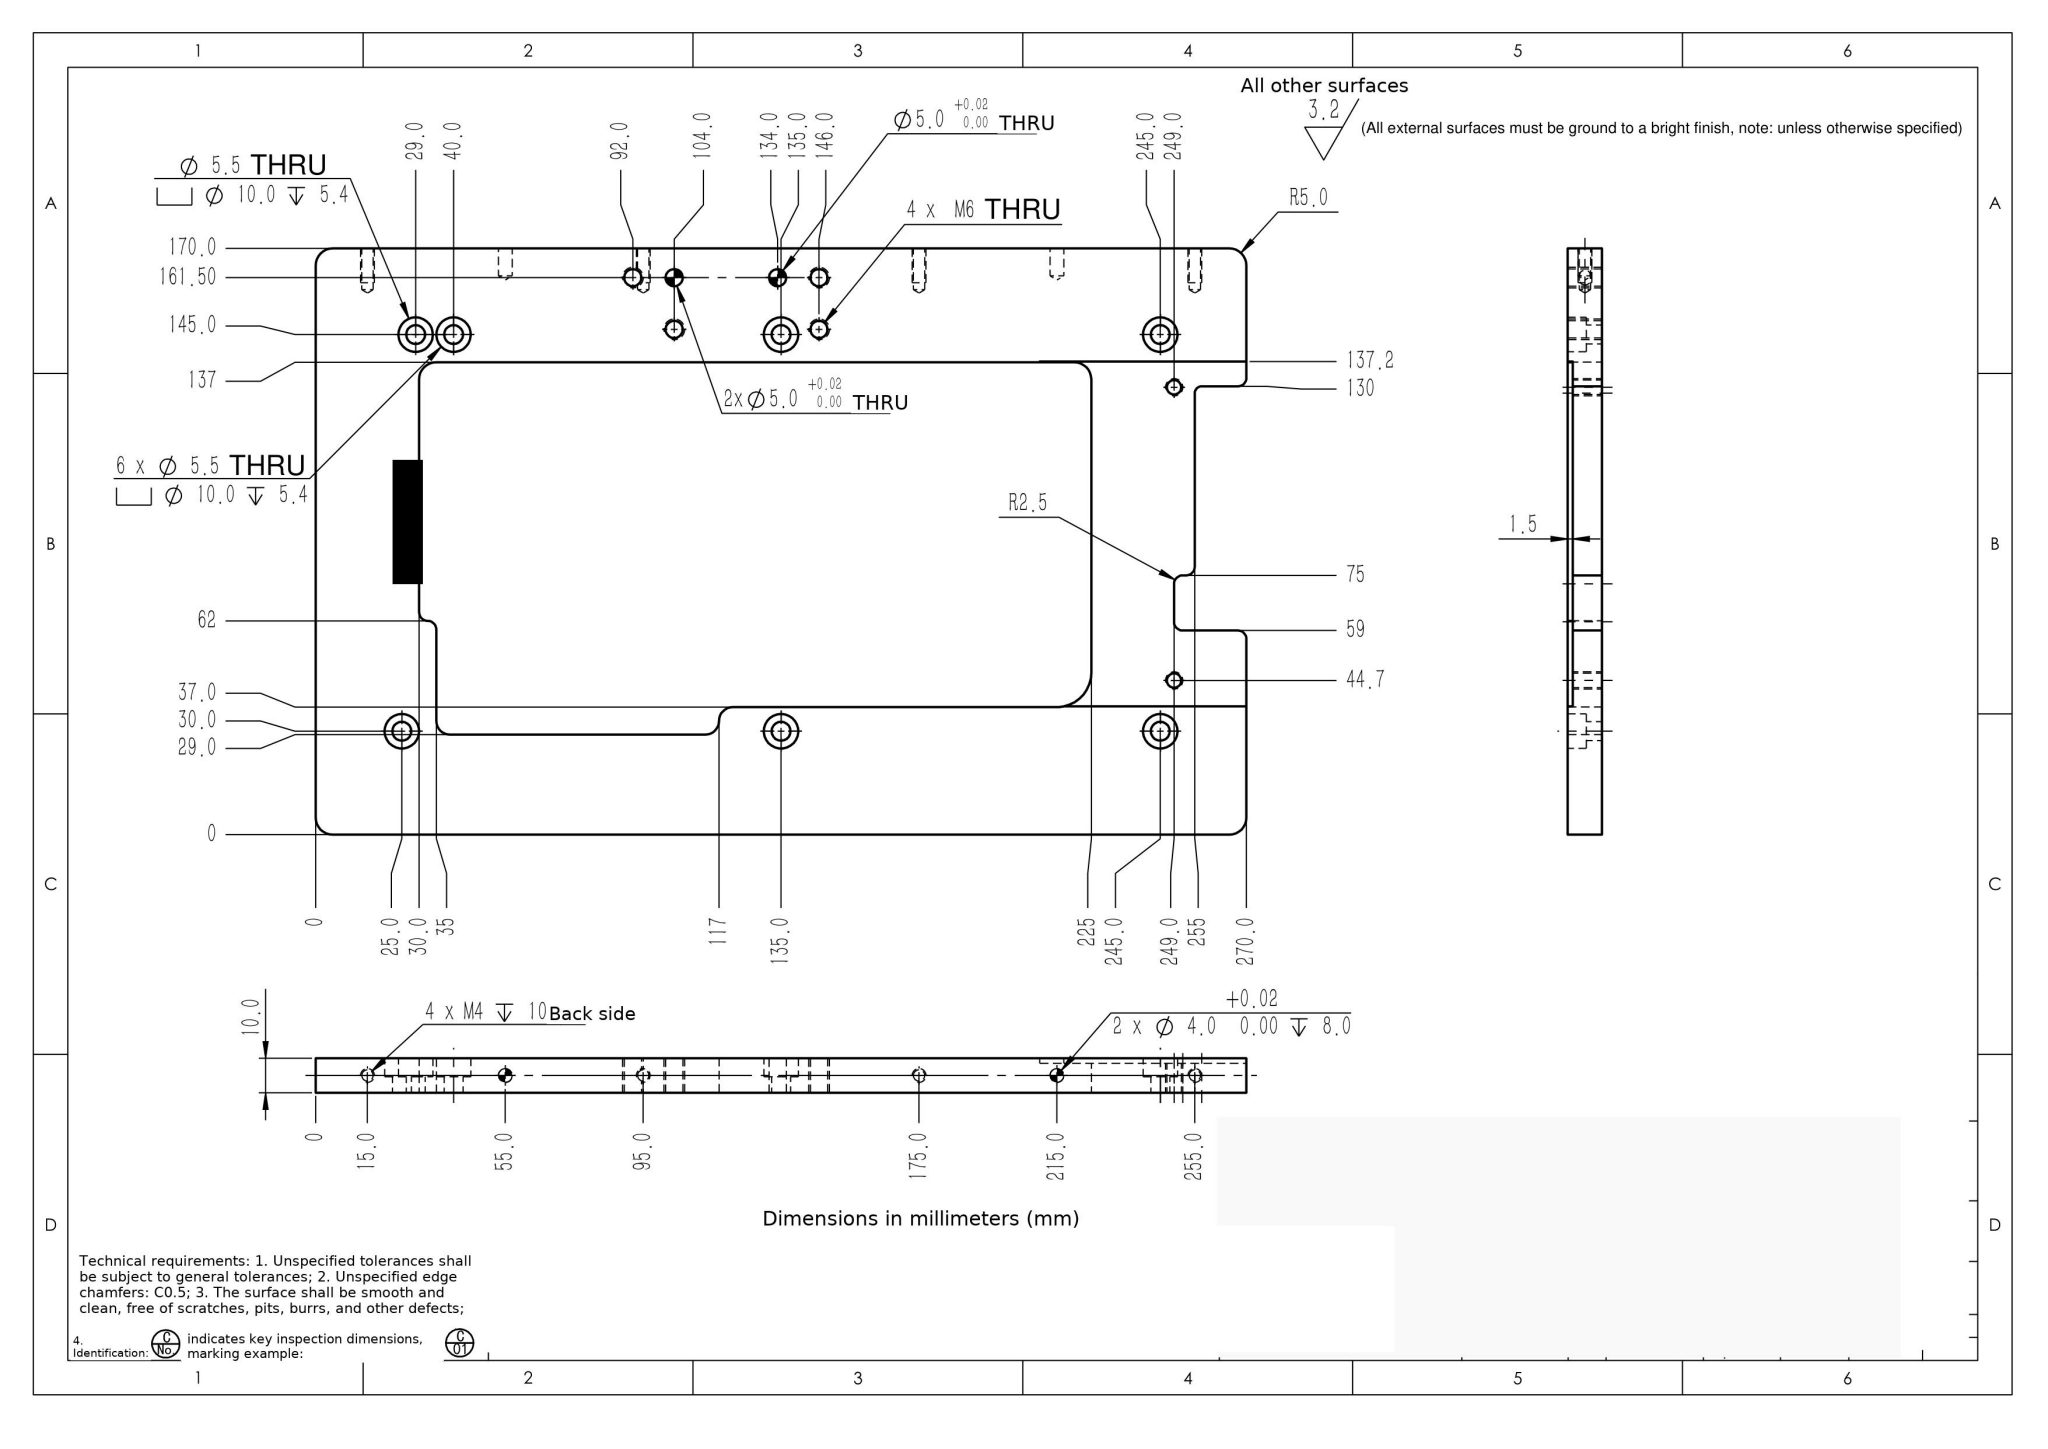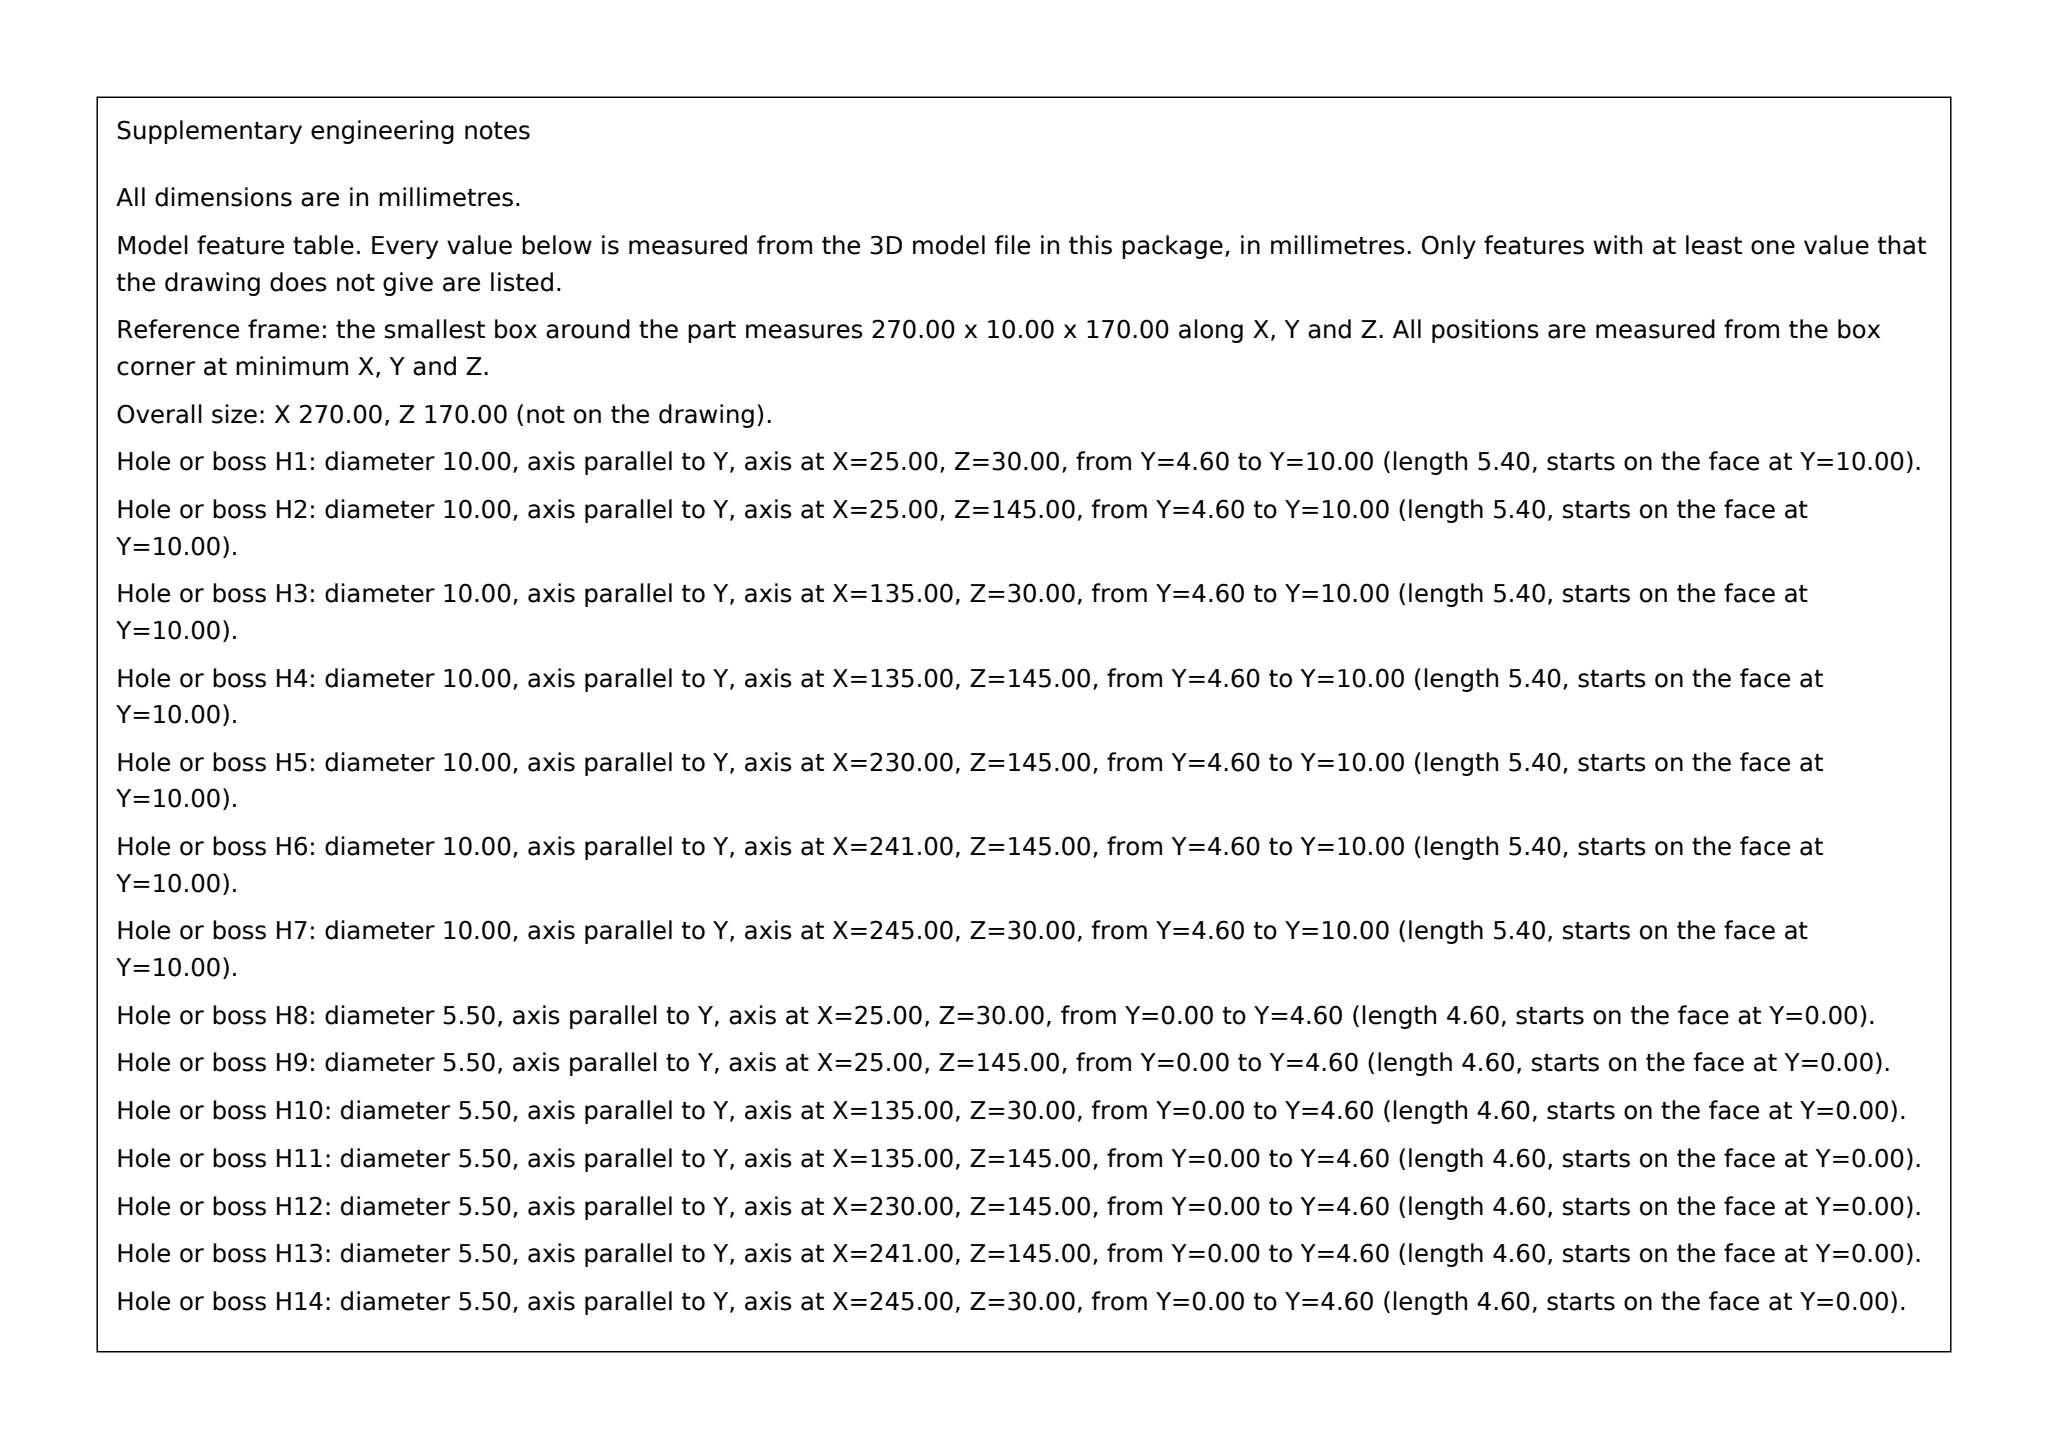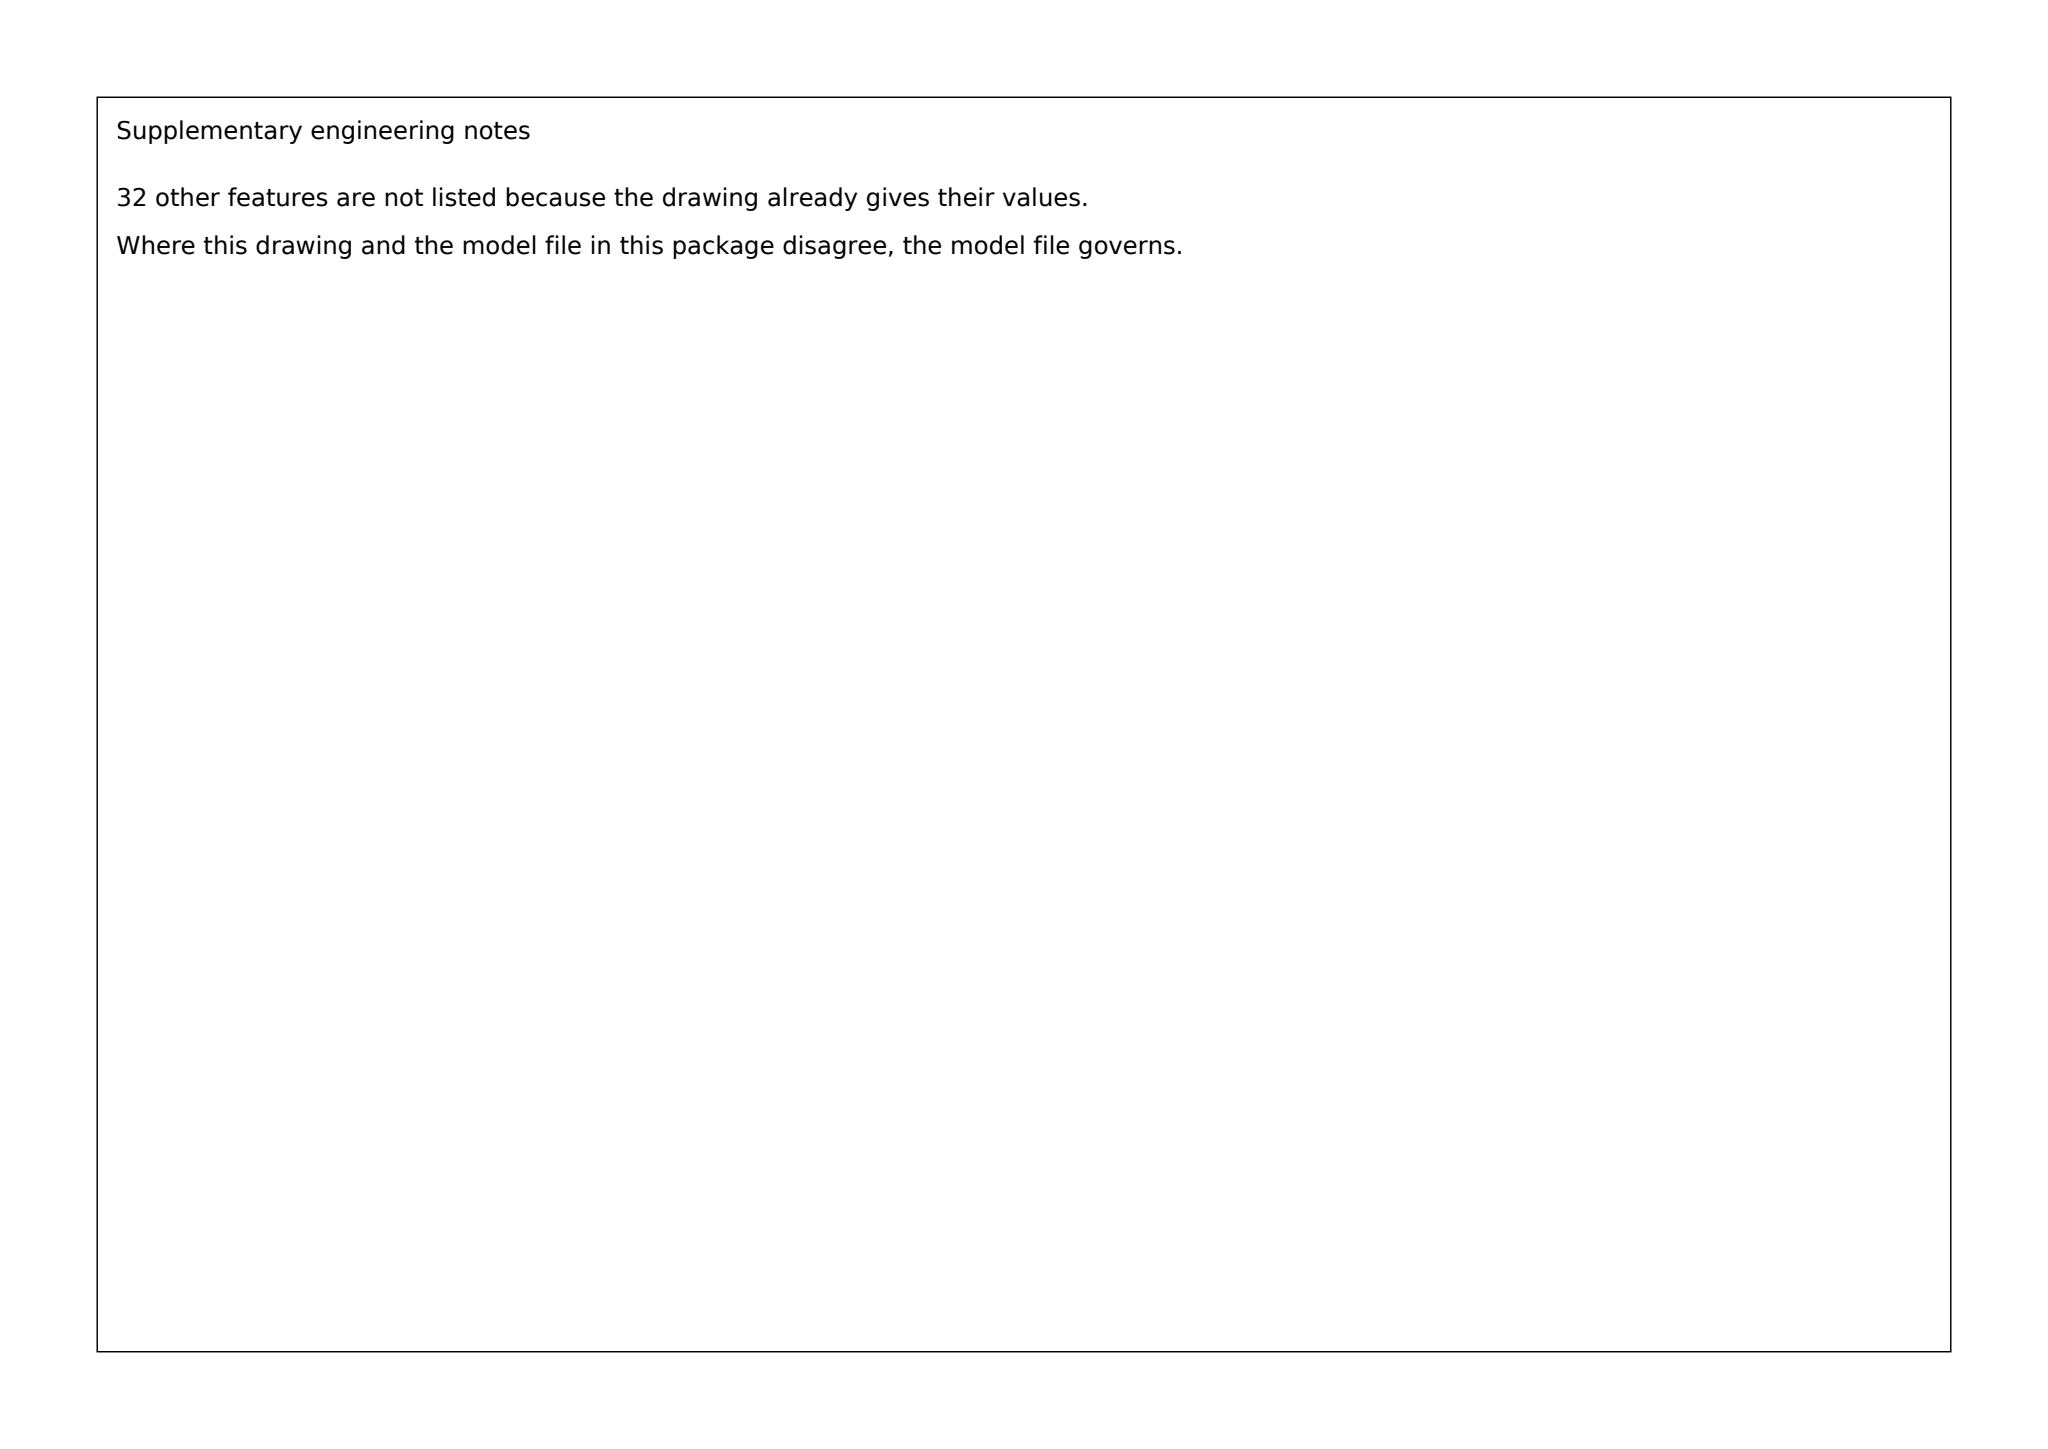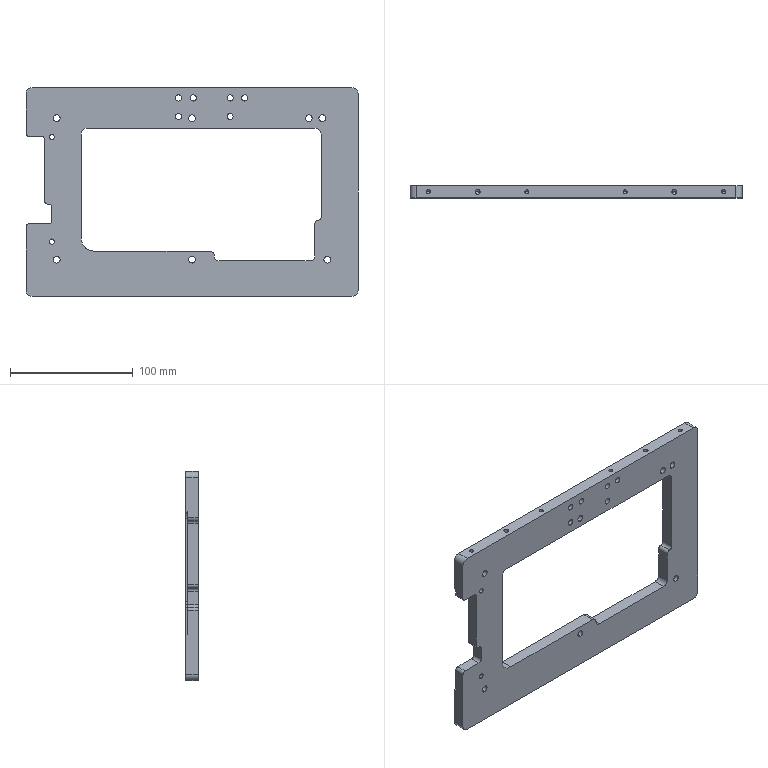Part | SolidWorks | mm | 1 solid | 123 faces | box 270 x 10 x 170 mm | volume 236419 mm3 | cylinder 74 | plane 37 | cone 12 | commonest cylinder face diameters 10 x20 5 x19 5.5 x14 3.3 x8 4 x5 4.2 x4 8 x3 20 x1